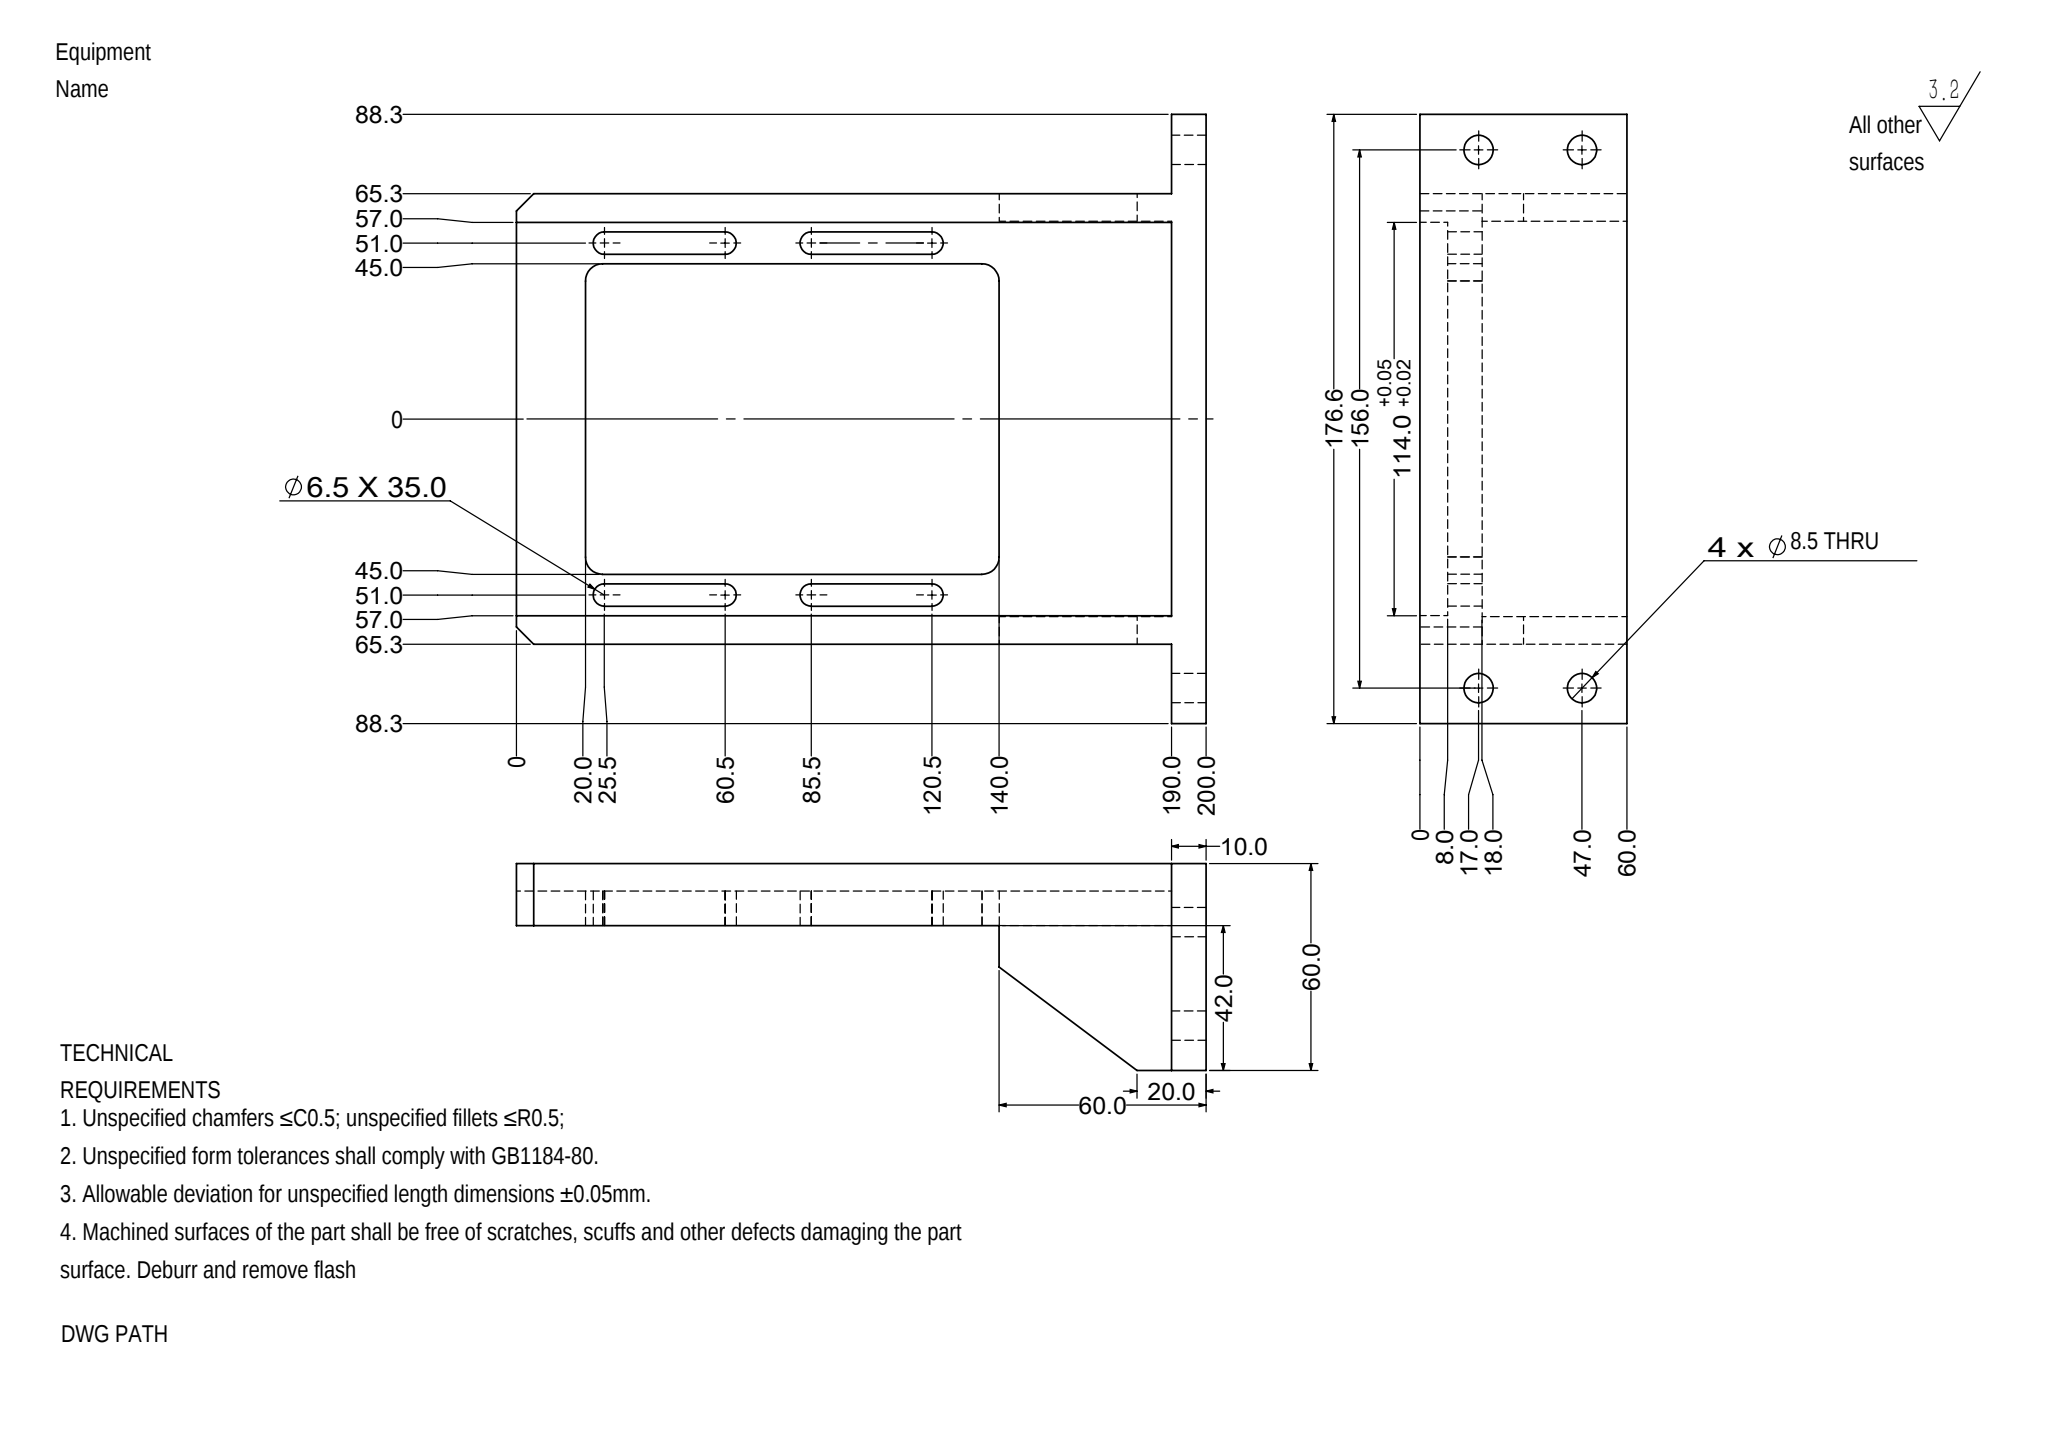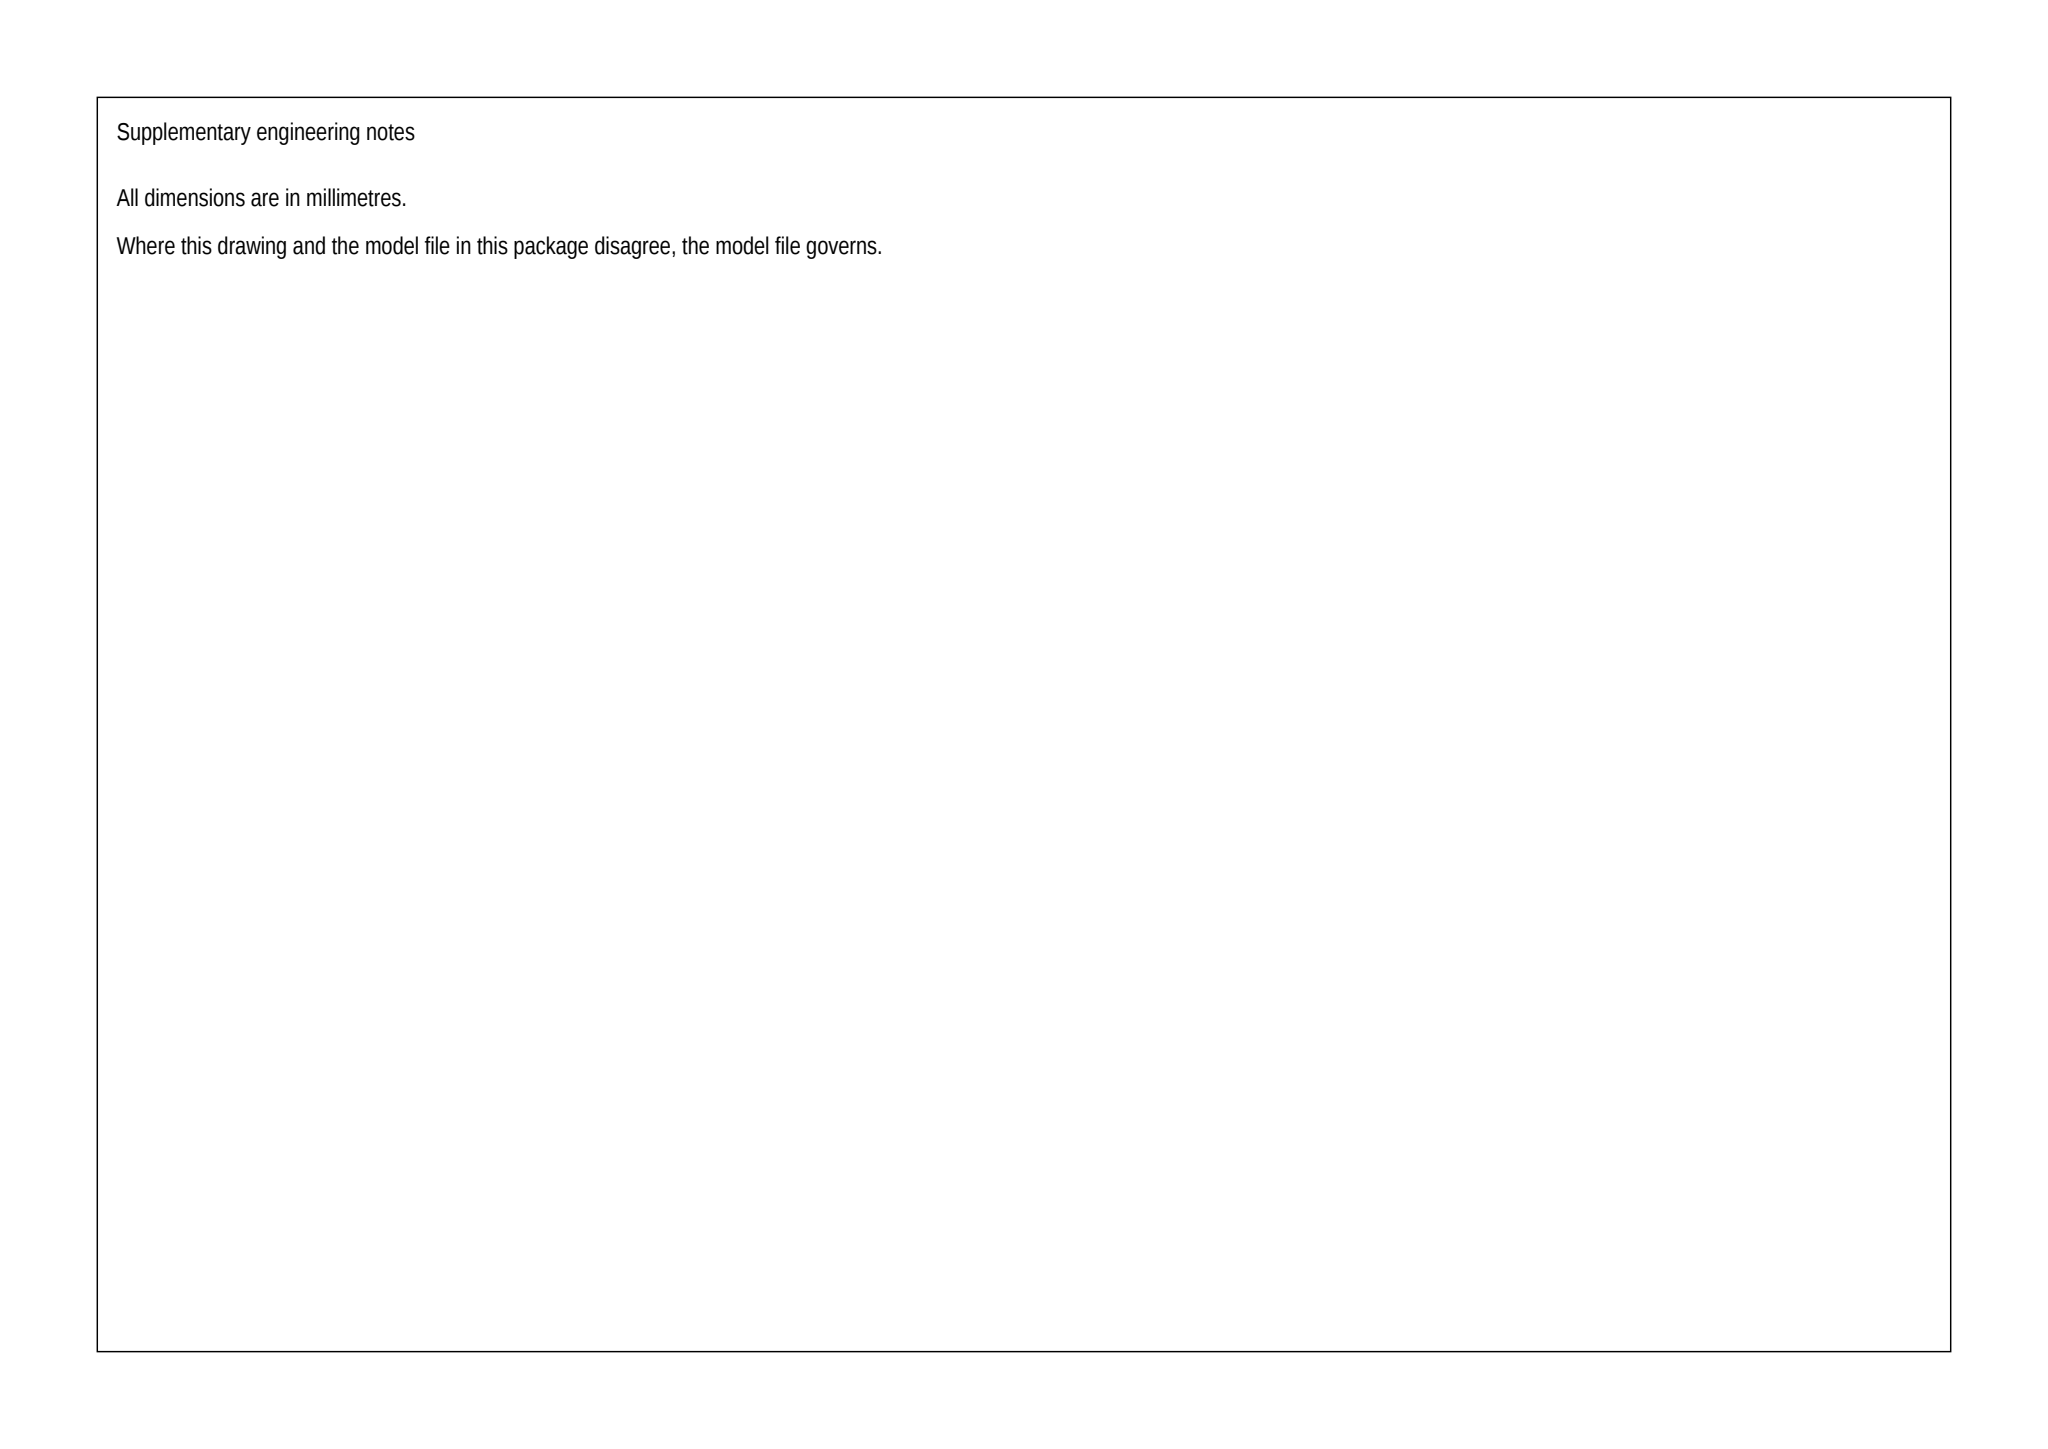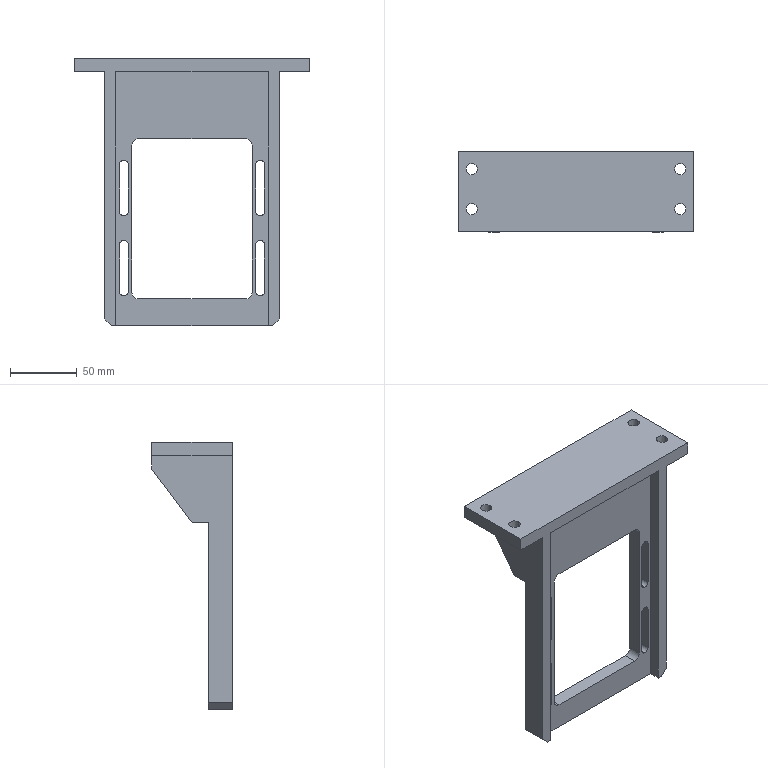Part | SolidWorks | mm | 1 solid | 64 faces | box 176.6 x 60 x 200 mm | volume 282399 mm3 | plane 36 | cylinder 28 | commonest cylinder face diameters 6.5 x16 8.5 x8 10 x4
Drawing notes:
CENTRAL POCKET 90 X 120, R5 CORNERS: THRU 10 THK | from the solid: pocket walls x 43.3-133.3 (90, ±45) and z 20.0-140.0 (120); 4 x Ø10 y-axis corner cyls at (48.3/128.3, 25.0/135.0) len 10.0 = R5; only y planes 8.0 & 18.0 -> 10 thk, through
FRONT VIEW: STEPPED END SECT 114.6 WIDE (57.3 EA SIDE OF CL) | from the solid: x-planes 31.0 and 145.6 (count 1 ea); CL at x=88.3 of 176.6 bbox => 57.3 ea side, 114.6 wide
STEPPED END SECT 8.0 LG FROM Z0 END FACE | from the solid: z=0 end face; step/chamfer transition at z=8.0 ahead of 65.3-wide sides (x=23.0/153.6)
STEP TRANSITION CHAM 8.0 X 8.0 EA SIDE (57.3 TO 65.3) | from the solid: half-width change 57.3 (x=31.0/145.6) to 65.3 (x=23.0/153.6) = 8.0 rise over 8.0 along Z
4X SLOT Ø6.5 X 35.0 C-C (41.5 OAL) THRU 10 THK PLATE | from the solid: Ø6.5 y-axis cyls L=10 at x=37.3 & 139.3, z=25.5/60.5 and 85.5/120.5 => 35.0 centres, 8 ends = 4 slots; plate y=8.0 to 18.0
2X CHAM 8 X 45 DEG AT 0 END: 114.6 W END TO 130.6 W BODY | from the solid: Side planes x=31.0/145.6 (114.6 W) blend to x=23.0/153.6 (130.6 W); x leg = 31.0-23.0 = 8.0 per side, no z-normal face between them (angled face at z=0 end)
W STEPS 130.6 TO 114.0 AT Z=140.0, 114.0 RUNS TO Z=190.0 | from the solid: z planes list 140.0 (3 faces: pocket end + 2 side steps) and 190.0; faces x=31.3/145.3 give 114.0 +0.05/+0.02 section ending at flange face z=190.0
END SECTION 114.6 W (57.3 EA SIDE OF CL) FROM Z=0 TO CHAM | from the solid: axis planes x=31.0 and x=145.6 -> 114.6 width, symmetric about x=88.3 (57.3 each side); end face at z=0.0
build123d program:
from build123d import *

# Parameters (mm, degrees)
SKETCH1_W                           = 176.6
SKETCH1_H                           = 60
BOSS_EXTRUDE1_DEPTH                 = 10
SKETCH3_W                           = 130.6
SKETCH3_H                           = 200
BOSS_EXTRUDE2_DEPTH                 = 18
SKETCH4_W                           = 8
SKETCH4_H                           = 42
BOSS_EXTRUDE3_DEPTH                 = 50
CHAMFER1_SIZE                       = 5
SKETCH6_W                           = 114
SKETCH6_H                           = 190
CUT_EXTRUDE3_DEPTH                  = 8
SKETCH7_W                           = 90
SKETCH7_H                           = 120
CUT_EXTRUDE4_DEPTH                  = 274.473
CUT_EXTRUDE6_DEPTH                  = 271.095
CUT_EXTRUDE9_DEPTH                  = 260.216
FILLET1_R                           = 5
F_8_5_8_5_DIAMETER_HOLE1_AT_2_COUNT = 2
F_8_5_8_5_DIAMETER_HOLE1_AT_2_PITCH = 30
CUT_EXTRUDE10_DEPTH                 = 272.83


with BuildPart() as part:
    # Sketch1 → Boss-Extrude1 (new body)
    with BuildSketch(Plane.XY):
        with Locations((88.3, 30)):
            Rectangle(SKETCH1_W, SKETCH1_H)
    extrude(amount=-BOSS_EXTRUDE1_DEPTH)

    # Sketch3 → Boss-Extrude2 (add)
    with BuildSketch(Plane.XZ):
        with Locations((88.3, -100)):
            Rectangle(SKETCH3_W, SKETCH3_H)
    extrude(amount=-BOSS_EXTRUDE2_DEPTH)

    # Sketch4 → Boss-Extrude3 (add)
    with BuildSketch(Plane(origin=(0, 0, -10), x_dir=(-1, 0, 0), z_dir=(0, 0, -1))):
        with Locations((-149.6, 39)):
            Rectangle(SKETCH4_W, SKETCH4_H)
        with Locations((-27, 39)):
            Rectangle(SKETCH4_W, SKETCH4_H)
    extrude(amount=BOSS_EXTRUDE3_DEPTH)

    # Chamfer1
    chamfer1_edges = [part.edges().sort_by_distance(p)[0] for p in [
        (23, 9, -200),
        (153.6, 9, -200),
    ]]
    chamfer(chamfer1_edges, length=CHAMFER1_SIZE)

    # Sketch6 → Cut-Extrude3 (cut)
    with BuildSketch(Plane.XZ):
        with Locations((88.3, -105)):
            Rectangle(SKETCH6_W, SKETCH6_H)
    extrude(amount=-CUT_EXTRUDE3_DEPTH, mode=Mode.SUBTRACT)

    # Sketch7 → Cut-Extrude4 (cut, through all)
    with BuildSketch(Plane.XZ):
        with Locations((88.3, -120)):
            Rectangle(SKETCH7_W, SKETCH7_H)
    extrude(amount=-CUT_EXTRUDE4_DEPTH, mode=Mode.SUBTRACT)

    # Sketch9 → Cut-Extrude6 (cut, through all)
    with BuildSketch(Plane(origin=(0, 18, 0), x_dir=(1, 0, 0), z_dir=(0, 1, 0))):
        with BuildLine():
            Line((142.55, 94.5), (142.55, 79.5))
            ThreePointArc((142.55, 79.5), (139.3, 76.25), (136.05, 79.5))
            Line((136.05, 79.5), (136.05, 94.5))
            ThreePointArc((136.05, 94.5), (139.3, 97.75), (142.55, 94.5))
        make_face()
        with BuildLine():
            Line((142.55, 154.5), (142.55, 139.5))
            ThreePointArc((142.55, 139.5), (139.3, 136.25), (136.05, 139.5))
            Line((136.05, 139.5), (136.05, 154.5))
            ThreePointArc((136.05, 154.5), (139.3, 157.75), (142.55, 154.5))
        make_face()
        with BuildLine():
            Line((34.05, 94.5), (34.05, 79.5))
            ThreePointArc((34.05, 79.5), (37.3, 76.25), (40.55, 79.5))
            Line((40.55, 79.5), (40.55, 94.5))
            ThreePointArc((40.55, 94.5), (37.3, 97.75), (34.05, 94.5))
        make_face()
        with BuildLine():
            Line((34.05, 154.5), (34.05, 139.5))
            ThreePointArc((34.05, 139.5), (37.3, 136.25), (40.55, 139.5))
            Line((40.55, 139.5), (40.55, 154.5))
            ThreePointArc((40.55, 154.5), (37.3, 157.75), (34.05, 154.5))
        make_face()
    extrude(amount=-CUT_EXTRUDE6_DEPTH, mode=Mode.SUBTRACT)

    # Sketch11 → Cut-Extrude9 (cut, through all)
    with BuildSketch(Plane(origin=(153.6, 0, 0), x_dir=(0, 0, -1), z_dir=(1, 0, 0))):
        Polygon((20, 60), (60, 30), (60, 60), align=None)
    extrude(amount=-CUT_EXTRUDE9_DEPTH, mode=Mode.SUBTRACT)

    # Fillet1
    fillet1_edges = [part.edges().sort_by_distance(p)[0] for p in [
        (133.3, 13, -60),
        (133.3, 13, -180),
        (43.3, 13, -180),
        (43.3, 13, -60),
    ]]
    fillet(fillet1_edges, radius=FILLET1_R)

    # Sketch13 → 8.5 _8.5_ Diameter Hole1 (revolve, cut)
    with BuildSketch(Plane(origin=(166.3, 47, 0), x_dir=(0, -1, 0), z_dir=(1, 0, 0))):
        Polygon((0, 0), (0, 12.654), (4.25, 10.1), (4.25, 0), align=None)
    f_8_5_8_5_diameter_hole1 = revolve(axis=Axis((166.3, 47, 6.35), (0, 0, -1)), mode=Mode.SUBTRACT)

    # 8.5 _8.5_ Diameter Hole1 at 2: 8.5 _8.5_ Diameter Hole1 ×2
    with Locations(*[(0, -i * F_8_5_8_5_DIAMETER_HOLE1_AT_2_PITCH, 0) for i in range(1, F_8_5_8_5_DIAMETER_HOLE1_AT_2_COUNT)]):
        add(f_8_5_8_5_diameter_hole1, mode=Mode.SUBTRACT)

    # Mirror1: 8.5 _8.5_ Diameter Hole1 across plane
    add(f_8_5_8_5_diameter_hole1.mirror(Plane(origin=(88.3, 0, 0), x_dir=(0, 0, 1), z_dir=(1, 0, 0))), mode=Mode.SUBTRACT)

    # Mirror1 copy 1 sketch → Mirror1 copy 1 (revolve, cut)
    with BuildSketch(Plane(origin=(10.3, 17, 0), x_dir=(0, -1, 0), z_dir=(-1, 0, 0))):
        Polygon((0, 0), (0, -12.654), (4.25, -10.1), (4.25, 0), align=None)
    revolve(axis=Axis((10.3, 17, 6.35), (0, 0, 1)), mode=Mode.SUBTRACT)

    # Sketch14 → Cut-Extrude10 (cut, through all)
    with BuildSketch(Plane.XZ.offset(-8)):
        with BuildLine():
            Line((40.55, -94.5), (40.55, -114.5))
            ThreePointArc((40.55, -114.5), (37.3, -117.75), (34.05, -114.5))
            Line((34.05, -114.5), (34.05, -94.5))
            ThreePointArc((34.05, -94.5), (37.3, -91.25), (40.55, -94.5))
        make_face()
        with BuildLine():
            Line((40.55, -154.5), (40.55, -174.5))
            ThreePointArc((40.55, -174.5), (37.3, -177.75), (34.05, -174.5))
            Line((34.05, -174.5), (34.05, -154.5))
            ThreePointArc((34.05, -154.5), (37.3, -151.25), (40.55, -154.5))
        make_face()
        with BuildLine():
            Line((142.55, -94.5), (142.55, -114.5))
            ThreePointArc((142.55, -114.5), (139.3, -117.75), (136.05, -114.5))
            Line((136.05, -114.5), (136.05, -94.5))
            ThreePointArc((136.05, -94.5), (139.3, -91.25), (142.55, -94.5))
        make_face()
        with BuildLine():
            Line((142.55, -154.5), (142.55, -174.5))
            ThreePointArc((142.55, -174.5), (139.3, -177.75), (136.05, -174.5))
            Line((136.05, -174.5), (136.05, -154.5))
            ThreePointArc((136.05, -154.5), (139.3, -151.25), (142.55, -154.5))
        make_face()
    extrude(amount=-CUT_EXTRUDE10_DEPTH, mode=Mode.SUBTRACT)


solid = part.part